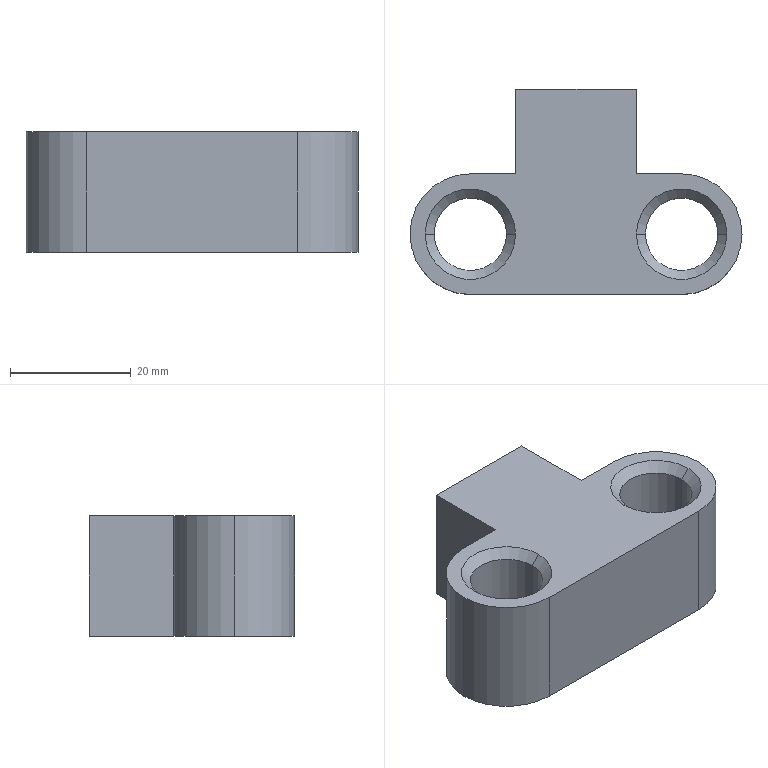Component | SolidWorks | ACQ40x30SB(0)+()-1_ZTDJ-L-400-04-24-MaterialPortBagClamp-T-shapedConnectingRod-2 | 1 solid | 27 faces | box 55 x 34 x 20 mm | volume 17034 mm3 | cone 10 | cylinder 9 | plane 8 | commonest cylinder face diameters 12 x4 20 x3 14 x2 | material 1023 Carbon Steel Sheet (SS)
build123d program:
from build123d import *

# Parameters (mm, degrees)
SKETCH1_R                  = 6
BOSS_EXTRUDE1_DEPTH        = 10
SKETCH4_W                  = 20
SKETCH4_H                  = 20
BOSS_EXTRUDE2_DEPTH        = 14
M14X1_5_TAPPED_HOLE1_D     = 14
M14X1_5_TAPPED_HOLE1_DEPTH = 25.5
M14X1_5_TAPPED_HOLE1_TIP   = 4.206
CHAMFER1_SIZE              = 1.5


with BuildPart() as part:
    # Sketch1 → Boss-Extrude1 (new, symmetric)
    with BuildSketch(Plane.XY):
        with BuildLine():
            Line((-17.5, 10), (17.5, 10))
            ThreePointArc((17.5, 10), (27.5, 0), (17.5, -10))
            Line((17.5, -10), (-17.5, -10))
            ThreePointArc((-17.5, -10), (-27.5, 0), (-17.5, 10))
        make_face()
        with Locations((17.5, 0)):
            Circle(SKETCH1_R, mode=Mode.SUBTRACT)
        with Locations((-17.5, 0)):
            Circle(SKETCH1_R, mode=Mode.SUBTRACT)
    extrude(amount=BOSS_EXTRUDE1_DEPTH, both=True)

    # Sketch4 → Boss-Extrude2 (add)
    with BuildSketch(Plane(origin=(0, 10, 0), x_dir=(1, 0, 0), z_dir=(0, 1, 0))):
        Rectangle(SKETCH4_W, SKETCH4_H)
    extrude(amount=BOSS_EXTRUDE2_DEPTH)

    # M14x1.5 Tapped Hole1
    with Locations(Plane(origin=(0, 24, 0), x_dir=(1, 0, 0), z_dir=(0, 1, 0))):
        with Locations((0, 0)):
            Hole(M14X1_5_TAPPED_HOLE1_D / 2, depth=M14X1_5_TAPPED_HOLE1_DEPTH)
            with Locations((0, 0, -(M14X1_5_TAPPED_HOLE1_DEPTH + M14X1_5_TAPPED_HOLE1_TIP / 2))):  # 118° drill point
                Cone(0, M14X1_5_TAPPED_HOLE1_D / 2, M14X1_5_TAPPED_HOLE1_TIP, mode=Mode.SUBTRACT)

    # Chamfer1
    chamfer1_edges = [part.edges().sort_by_distance(p)[0] for p in [
        (11.5, 0, -10),
        (11.5, 0, 10),
        (-23.5, 0, -10),
        (-23.5, 0, 10),
    ]]
    chamfer(chamfer1_edges, length=CHAMFER1_SIZE)


solid = part.part

# Placed as in the assembly
solid = solid.moved(Location((-28.439, -84.245, 290), (0, 0, 0)))
STEP:
#1=COLOUR_RGB('',0.7922,0.8196,0.9333);
#2=FILL_AREA_STYLE_COLOUR('',#1);
#3=FILL_AREA_STYLE('',(#2));
#4=SURFACE_STYLE_FILL_AREA(#3);
#5=SURFACE_SIDE_STYLE('',(#4));
#6=SURFACE_STYLE_USAGE(.BOTH.,#5);
#7=PRESENTATION_STYLE_ASSIGNMENT((#6));
#8=CARTESIAN_POINT('',(-0.6669,-3.317,11.752));
#9=VERTEX_POINT('',#8);
#10=CARTESIAN_POINT('',(-0.1944,-3.317,11.752));
#11=VERTEX_POINT('',#10);
#12=CARTESIAN_POINT('',(-0.4307,-3.317,11.752));
#13=DIRECTION('',(0.,0.,1.));
#14=DIRECTION('',(1.,0.,0.));
#15=AXIS2_PLACEMENT_3D('',#12,#13,#14);
#16=CIRCLE('',#15,0.2362);
#17=EDGE_CURVE('',#9,#11,#16,.T.);
#18=ORIENTED_EDGE('',*,*,#17,.F.);
#19=CARTESIAN_POINT('',(-0.7259,-3.317,11.811));
#20=VERTEX_POINT('',#19);
#21=CARTESIAN_POINT('',(-0.6669,-3.317,11.752));
#22=DIRECTION('',(-0.7071,0.,0.7071));
#23=VECTOR('',#22,39.37);
#24=LINE('',#21,#23);
#25=EDGE_CURVE('',#9,#20,#24,.T.);
#26=ORIENTED_EDGE('',*,*,#25,.T.);
#27=CARTESIAN_POINT('',(-0.1354,-3.317,11.811));
#28=VERTEX_POINT('',#27);
#29=CARTESIAN_POINT('',(-0.4307,-3.317,11.811));
#30=DIRECTION('',(0.,0.,-1.));
#31=DIRECTION('',(1.,0.,0.));
#32=AXIS2_PLACEMENT_3D('',#29,#30,#31);
#33=CIRCLE('',#32,0.2953);
#34=EDGE_CURVE('',#28,#20,#33,.T.);
#35=ORIENTED_EDGE('',*,*,#34,.F.);
#36=CARTESIAN_POINT('',(-0.1944,-3.317,11.752));
#37=DIRECTION('',(0.7071,0.,0.7071));
#38=VECTOR('',#37,39.37);
#39=LINE('',#36,#38);
#40=EDGE_CURVE('',#11,#28,#39,.T.);
#41=ORIENTED_EDGE('',*,*,#40,.F.);
#42=EDGE_LOOP('',(#18,#26,#35,#41));
#43=FACE_OUTER_BOUND('',#42,.T.);
#44=CARTESIAN_POINT('',(-0.4307,-3.317,11.752));
#45=DIRECTION('',(0.,0.,1.));
#46=DIRECTION('',(1.,0.,0.));
#47=AXIS2_PLACEMENT_3D('',#44,#45,#46);
#48=CONICAL_SURFACE('',#47,0.2362,0.7854);
#49=ADVANCED_FACE('',(#43),#48,.F.);
#50=CARTESIAN_POINT('',(-2.045,-3.317,11.752));
#51=VERTEX_POINT('',#50);
#52=CARTESIAN_POINT('',(-1.572,-3.317,11.752));
#53=VERTEX_POINT('',#52);
#54=CARTESIAN_POINT('',(-1.809,-3.317,11.752));
#55=DIRECTION('',(0.,0.,1.));
#56=DIRECTION('',(1.,0.,0.));
#57=AXIS2_PLACEMENT_3D('',#54,#55,#56);
#58=CIRCLE('',#57,0.2362);
#59=EDGE_CURVE('',#51,#53,#58,.T.);
#60=ORIENTED_EDGE('',*,*,#59,.F.);
#61=CARTESIAN_POINT('',(-2.104,-3.317,11.811));
#62=VERTEX_POINT('',#61);
#63=CARTESIAN_POINT('',(-2.045,-3.317,11.752));
#64=DIRECTION('',(-0.7071,0.,0.7071));
#65=VECTOR('',#64,39.37);
#66=LINE('',#63,#65);
#67=EDGE_CURVE('',#51,#62,#66,.T.);
#68=ORIENTED_EDGE('',*,*,#67,.T.);
#69=CARTESIAN_POINT('',(-1.513,-3.317,11.811));
#70=VERTEX_POINT('',#69);
#71=CARTESIAN_POINT('',(-1.809,-3.317,11.811));
#72=DIRECTION('',(0.,0.,-1.));
#73=DIRECTION('',(1.,0.,0.));
#74=AXIS2_PLACEMENT_3D('',#71,#72,#73);
#75=CIRCLE('',#74,0.2953);
#76=EDGE_CURVE('',#70,#62,#75,.T.);
#77=ORIENTED_EDGE('',*,*,#76,.F.);
#78=CARTESIAN_POINT('',(-1.572,-3.317,11.752));
#79=DIRECTION('',(0.7071,0.,0.7071));
#80=VECTOR('',#79,39.37);
#81=LINE('',#78,#80);
#82=EDGE_CURVE('',#53,#70,#81,.T.);
#83=ORIENTED_EDGE('',*,*,#82,.F.);
#84=EDGE_LOOP('',(#60,#68,#77,#83));
#85=FACE_OUTER_BOUND('',#84,.T.);
#86=CARTESIAN_POINT('',(-1.809,-3.317,11.752));
#87=DIRECTION('',(0.,0.,1.));
#88=DIRECTION('',(1.,0.,0.));
#89=AXIS2_PLACEMENT_3D('',#86,#87,#88);
#90=CONICAL_SURFACE('',#89,0.2362,0.7854);
#91=ADVANCED_FACE('',(#85),#90,.F.);
#92=CARTESIAN_POINT('',(-0.1944,-3.317,11.083));
#93=VERTEX_POINT('',#92);
#94=CARTESIAN_POINT('',(-0.6669,-3.317,11.083));
#95=VERTEX_POINT('',#94);
#96=CARTESIAN_POINT('',(-0.4307,-3.317,11.083));
#97=DIRECTION('',(0.,0.,-1.));
#98=DIRECTION('',(1.,0.,0.));
#99=AXIS2_PLACEMENT_3D('',#96,#97,#98);
#100=CIRCLE('',#99,0.2362);
#101=EDGE_CURVE('',#93,#95,#100,.T.);
#102=ORIENTED_EDGE('',*,*,#101,.F.);
#103=CARTESIAN_POINT('',(-0.1354,-3.317,11.024));
#104=VERTEX_POINT('',#103);
#105=CARTESIAN_POINT('',(-0.1354,-3.317,11.024));
#106=DIRECTION('',(0.7071,0.,-0.7071));
#107=VECTOR('',#106,39.37);
#108=LINE('',#105,#107);
#109=EDGE_CURVE('',#93,#104,#108,.T.);
#110=ORIENTED_EDGE('',*,*,#109,.T.);
#111=CARTESIAN_POINT('',(-0.7259,-3.317,11.024));
#112=VERTEX_POINT('',#111);
#113=CARTESIAN_POINT('',(-0.4307,-3.317,11.024));
#114=DIRECTION('',(0.,0.,1.));
#115=DIRECTION('',(1.,0.,0.));
#116=AXIS2_PLACEMENT_3D('',#113,#114,#115);
#117=CIRCLE('',#116,0.2953);
#118=EDGE_CURVE('',#112,#104,#117,.T.);
#119=ORIENTED_EDGE('',*,*,#118,.F.);
#120=CARTESIAN_POINT('',(-0.7259,-3.317,11.024));
#121=DIRECTION('',(-0.7071,0.,-0.7071));
#122=VECTOR('',#121,39.37);
#123=LINE('',#120,#122);
#124=EDGE_CURVE('',#95,#112,#123,.T.);
#125=ORIENTED_EDGE('',*,*,#124,.F.);
#126=EDGE_LOOP('',(#102,#110,#119,#125));
#127=FACE_OUTER_BOUND('',#126,.T.);
#128=CARTESIAN_POINT('',(-0.4307,-3.317,11.024));
#129=DIRECTION('',(0.,0.,-1.));
#130=DIRECTION('',(-1.,0.,0.));
#131=AXIS2_PLACEMENT_3D('',#128,#129,#130);
#132=CONICAL_SURFACE('',#131,0.2953,0.7854);
#133=ADVANCED_FACE('',(#127),#132,.F.);
#134=CARTESIAN_POINT('',(-1.572,-3.317,11.083));
#135=VERTEX_POINT('',#134);
#136=CARTESIAN_POINT('',(-2.045,-3.317,11.083));
#137=VERTEX_POINT('',#136);
#138=CARTESIAN_POINT('',(-1.809,-3.317,11.083));
#139=DIRECTION('',(0.,0.,-1.));
#140=DIRECTION('',(1.,0.,0.));
#141=AXIS2_PLACEMENT_3D('',#138,#139,#140);
#142=CIRCLE('',#141,0.2362);
#143=EDGE_CURVE('',#135,#137,#142,.T.);
#144=ORIENTED_EDGE('',*,*,#143,.F.);
#145=CARTESIAN_POINT('',(-1.513,-3.317,11.024));
#146=VERTEX_POINT('',#145);
#147=CARTESIAN_POINT('',(-1.513,-3.317,11.024));
#148=DIRECTION('',(0.7071,0.,-0.7071));
#149=VECTOR('',#148,39.37);
#150=LINE('',#147,#149);
#151=EDGE_CURVE('',#135,#146,#150,.T.);
#152=ORIENTED_EDGE('',*,*,#151,.T.);
#153=CARTESIAN_POINT('',(-2.104,-3.317,11.024));
#154=VERTEX_POINT('',#153);
#155=CARTESIAN_POINT('',(-1.809,-3.317,11.024));
#156=DIRECTION('',(0.,0.,1.));
#157=DIRECTION('',(1.,0.,0.));
#158=AXIS2_PLACEMENT_3D('',#155,#156,#157);
#159=CIRCLE('',#158,0.2953);
#160=EDGE_CURVE('',#154,#146,#159,.T.);
#161=ORIENTED_EDGE('',*,*,#160,.F.);
#162=CARTESIAN_POINT('',(-2.104,-3.317,11.024));
#163=DIRECTION('',(-0.7071,0.,-0.7071));
#164=VECTOR('',#163,39.37);
#165=LINE('',#162,#164);
#166=EDGE_CURVE('',#137,#154,#165,.T.);
#167=ORIENTED_EDGE('',*,*,#166,.F.);
#168=EDGE_LOOP('',(#144,#152,#161,#167));
#169=FACE_OUTER_BOUND('',#168,.T.);
#170=CARTESIAN_POINT('',(-1.809,-3.317,11.024));
#171=DIRECTION('',(0.,0.,-1.));
#172=DIRECTION('',(-1.,0.,0.));
#173=AXIS2_PLACEMENT_3D('',#170,#171,#172);
#174=CONICAL_SURFACE('',#173,0.2953,0.7854);
#175=ADVANCED_FACE('',(#169),#174,.F.);
#176=CARTESIAN_POINT('',(-1.12,-3.376,11.142));
#177=VERTEX_POINT('',#176);
#178=CARTESIAN_POINT('',(-1.12,-3.376,11.693));
#179=VERTEX_POINT('',#178);
#180=CARTESIAN_POINT('',(-1.12,-3.376,11.417));
#181=DIRECTION('',(0.,1.,0.));
#182=DIRECTION('',(0.,0.,1.));
#183=AXIS2_PLACEMENT_3D('',#180,#181,#182);
#184=CIRCLE('',#183,0.2756);
#185=EDGE_CURVE('',#177,#179,#184,.T.);
#186=ORIENTED_EDGE('',*,*,#185,.F.);
#187=CARTESIAN_POINT('',(-1.12,-2.372,11.142));
#188=VERTEX_POINT('',#187);
#189=CARTESIAN_POINT('',(-1.12,-2.372,11.142));
#190=DIRECTION('',(0.,1.,0.));
#191=VECTOR('',#190,39.37);
#192=LINE('',#189,#191);
#193=EDGE_CURVE('',#177,#188,#192,.T.);
#194=ORIENTED_EDGE('',*,*,#193,.T.);
#195=CARTESIAN_POINT('',(-1.12,-2.372,11.693));
#196=VERTEX_POINT('',#195);
#197=CARTESIAN_POINT('',(-1.12,-2.372,11.417));
#198=DIRECTION('',(0.,1.,0.));
#199=DIRECTION('',(0.,0.,1.));
#200=AXIS2_PLACEMENT_3D('',#197,#198,#199);
#201=CIRCLE('',#200,0.2756);
#202=EDGE_CURVE('',#188,#196,#201,.T.);
#203=ORIENTED_EDGE('',*,*,#202,.T.);
#204=CARTESIAN_POINT('',(-1.12,-2.372,11.693));
#205=DIRECTION('',(0.,1.,0.));
#206=VECTOR('',#205,39.37);
#207=LINE('',#204,#206);
#208=EDGE_CURVE('',#179,#196,#207,.T.);
#209=ORIENTED_EDGE('',*,*,#208,.F.);
#210=EDGE_LOOP('',(#186,#194,#203,#209));
#211=FACE_OUTER_BOUND('',#210,.T.);
#212=CARTESIAN_POINT('',(-1.12,-2.372,11.417));
#213=DIRECTION('',(0.,1.,0.));
#214=DIRECTION('',(0.,0.,1.));
#215=AXIS2_PLACEMENT_3D('',#212,#213,#214);
#216=CYLINDRICAL_SURFACE('',#215,0.2756);
#217=ADVANCED_FACE('',(#211),#216,.F.);
#218=CARTESIAN_POINT('',(-1.12,-3.541,11.417));
#219=VERTEX_POINT('',#218);
#220=CARTESIAN_POINT('',(-1.12,-3.376,11.693));
#221=DIRECTION('',(0.,0.515,0.8572));
#222=VECTOR('',#221,39.37);
#223=LINE('',#220,#222);
#224=EDGE_CURVE('',#219,#179,#223,.T.);
#225=ORIENTED_EDGE('',*,*,#224,.F.);
#226=CARTESIAN_POINT('',(-1.12,-3.376,11.142));
#227=DIRECTION('',(0.,0.515,-0.8572));
#228=VECTOR('',#227,39.37);
#229=LINE('',#226,#228);
#230=EDGE_CURVE('',#219,#177,#229,.T.);
#231=ORIENTED_EDGE('',*,*,#230,.T.);
#232=ORIENTED_EDGE('',*,*,#185,.T.);
#233=EDGE_LOOP('',(#225,#231,#232));
#234=FACE_OUTER_BOUND('',#233,.T.);
#235=CARTESIAN_POINT('',(-1.12,-3.376,11.417));
#236=DIRECTION('',(0.,1.,0.));
#237=DIRECTION('',(0.,0.,1.));
#238=AXIS2_PLACEMENT_3D('',#235,#236,#237);
#239=CONICAL_SURFACE('',#238,0.2756,1.03);
#240=ADVANCED_FACE('',(#234),#239,.F.);
#241=ORIENTED_EDGE('',*,*,#59,.T.);
#242=CARTESIAN_POINT('',(-1.572,-3.317,11.811));
#243=DIRECTION('',(0.,0.,-1.));
#244=VECTOR('',#243,39.37);
#245=LINE('',#242,#244);
#246=EDGE_CURVE('',#53,#135,#245,.T.);
#247=ORIENTED_EDGE('',*,*,#246,.T.);
#248=ORIENTED_EDGE('',*,*,#143,.T.);
#249=CARTESIAN_POINT('',(-2.045,-3.317,11.811));
#250=DIRECTION('',(0.,0.,-1.));
#251=VECTOR('',#250,39.37);
#252=LINE('',#249,#251);
#253=EDGE_CURVE('',#51,#137,#252,.T.);
#254=ORIENTED_EDGE('',*,*,#253,.F.);
#255=EDGE_LOOP('',(#241,#247,#248,#254));
#256=FACE_OUTER_BOUND('',#255,.T.);
#257=CARTESIAN_POINT('',(-1.809,-3.317,11.811));
#258=DIRECTION('',(0.,0.,-1.));
#259=DIRECTION('',(-1.,0.,0.));
#260=AXIS2_PLACEMENT_3D('',#257,#258,#259);
#261=CYLINDRICAL_SURFACE('',#260,0.2362);
#262=ADVANCED_FACE('',(#256),#261,.F.);
#263=ORIENTED_EDGE('',*,*,#17,.T.);
#264=CARTESIAN_POINT('',(-0.1944,-3.317,11.811));
#265=DIRECTION('',(0.,0.,-1.));
#266=VECTOR('',#265,39.37);
#267=LINE('',#264,#266);
#268=EDGE_CURVE('',#11,#93,#267,.T.);
#269=ORIENTED_EDGE('',*,*,#268,.T.);
#270=ORIENTED_EDGE('',*,*,#101,.T.);
#271=CARTESIAN_POINT('',(-0.6669,-3.317,11.811));
#272=DIRECTION('',(0.,0.,-1.));
#273=VECTOR('',#272,39.37);
#274=LINE('',#271,#273);
#275=EDGE_CURVE('',#9,#95,#274,.T.);
#276=ORIENTED_EDGE('',*,*,#275,.F.);
#277=EDGE_LOOP('',(#263,#269,#270,#276));
#278=FACE_OUTER_BOUND('',#277,.T.);
#279=CARTESIAN_POINT('',(-0.4307,-3.317,11.811));
#280=DIRECTION('',(0.,0.,-1.));
#281=DIRECTION('',(-1.,0.,0.));
#282=AXIS2_PLACEMENT_3D('',#279,#280,#281);
#283=CYLINDRICAL_SURFACE('',#282,0.2362);
#284=ADVANCED_FACE('',(#278),#283,.F.);
#285=CARTESIAN_POINT('',(-2.202,-3.317,11.811));
#286=VERTEX_POINT('',#285);
#287=CARTESIAN_POINT('',(-1.809,-3.71,11.811));
#288=VERTEX_POINT('',#287);
#289=CARTESIAN_POINT('',(-1.809,-3.317,11.811));
#290=DIRECTION('',(0.,0.,1.));
#291=DIRECTION('',(1.,0.,0.));
#292=AXIS2_PLACEMENT_3D('',#289,#290,#291);
#293=CIRCLE('',#292,0.3937);
#294=EDGE_CURVE('',#286,#288,#293,.T.);
#295=ORIENTED_EDGE('',*,*,#294,.F.);
#296=CARTESIAN_POINT('',(-2.202,-3.317,11.024));
#297=VERTEX_POINT('',#296);
#298=CARTESIAN_POINT('',(-2.202,-3.317,11.811));
#299=DIRECTION('',(0.,0.,-1.));
#300=VECTOR('',#299,39.37);
#301=LINE('',#298,#300);
#302=EDGE_CURVE('',#286,#297,#301,.T.);
#303=ORIENTED_EDGE('',*,*,#302,.T.);
#304=CARTESIAN_POINT('',(-1.809,-3.71,11.024));
#305=VERTEX_POINT('',#304);
#306=CARTESIAN_POINT('',(-1.809,-3.317,11.024));
#307=DIRECTION('',(0.,0.,1.));
#308=DIRECTION('',(1.,0.,0.));
#309=AXIS2_PLACEMENT_3D('',#306,#307,#308);
#310=CIRCLE('',#309,0.3937);
#311=EDGE_CURVE('',#297,#305,#310,.T.);
#312=ORIENTED_EDGE('',*,*,#311,.T.);
#313=CARTESIAN_POINT('',(-1.809,-3.71,11.811));
#314=DIRECTION('',(0.,0.,-1.));
#315=VECTOR('',#314,39.37);
#316=LINE('',#313,#315);
#317=EDGE_CURVE('',#288,#305,#316,.T.);
#318=ORIENTED_EDGE('',*,*,#317,.F.);
#319=EDGE_LOOP('',(#295,#303,#312,#318));
#320=FACE_OUTER_BOUND('',#319,.T.);
#321=CARTESIAN_POINT('',(-1.809,-3.317,11.811));
#322=DIRECTION('',(0.,0.,-1.));
#323=DIRECTION('',(-1.,0.,0.));
#324=AXIS2_PLACEMENT_3D('',#321,#322,#323);
#325=CYLINDRICAL_SURFACE('',#324,0.3937);
#326=ADVANCED_FACE('',(#320),#325,.T.);
#327=CARTESIAN_POINT('',(-0.7259,-2.923,11.811));
#328=VERTEX_POINT('',#327);
#329=CARTESIAN_POINT('',(-0.7259,-2.923,11.024));
#330=VERTEX_POINT('',#329);
#331=CARTESIAN_POINT('',(-0.7259,-2.923,11.811));
#332=DIRECTION('',(0.,0.,-1.));
#333=VECTOR('',#332,39.37);
#334=LINE('',#331,#333);
#335=EDGE_CURVE('',#328,#330,#334,.T.);
#336=ORIENTED_EDGE('',*,*,#335,.F.);
#337=CARTESIAN_POINT('',(-0.4307,-2.923,11.811));
#338=VERTEX_POINT('',#337);
#339=CARTESIAN_POINT('',(-1.809,-2.923,11.811));
#340=DIRECTION('',(-1.,-0.,0.));
#341=VECTOR('',#340,39.37);
#342=LINE('',#339,#341);
#343=EDGE_CURVE('',#338,#328,#342,.T.);
#344=ORIENTED_EDGE('',*,*,#343,.F.);
#345=CARTESIAN_POINT('',(-0.4307,-2.923,11.024));
#346=VERTEX_POINT('',#345);
#347=CARTESIAN_POINT('',(-0.4307,-2.923,11.811));
#348=DIRECTION('',(0.,0.,-1.));
#349=VECTOR('',#348,39.37);
#350=LINE('',#347,#349);
#351=EDGE_CURVE('',#338,#346,#350,.T.);
#352=ORIENTED_EDGE('',*,*,#351,.T.);
#353=CARTESIAN_POINT('',(-1.809,-2.923,11.024));
#354=DIRECTION('',(-1.,-0.,0.));
#355=VECTOR('',#354,39.37);
#356=LINE('',#353,#355);
#357=EDGE_CURVE('',#346,#330,#356,.T.);
#358=ORIENTED_EDGE('',*,*,#357,.T.);
#359=EDGE_LOOP('',(#336,#344,#352,#358));
#360=FACE_OUTER_BOUND('',#359,.T.);
#361=CARTESIAN_POINT('',(-1.809,-2.923,11.811));
#362=DIRECTION('',(0.,-1.,0.));
#363=DIRECTION('',(1.,0.,0.));
#364=AXIS2_PLACEMENT_3D('',#361,#362,#363);
#365=PLANE('',#364);
#366=ADVANCED_FACE('',(#360),#365,.F.);
#367=CARTESIAN_POINT('',(-1.513,-2.923,11.024));
#368=VERTEX_POINT('',#367);
#369=CARTESIAN_POINT('',(-1.513,-2.923,11.811));
#370=VERTEX_POINT('',#369);
#371=CARTESIAN_POINT('',(-1.513,-2.923,11.811));
#372=DIRECTION('',(0.,0.,1.));
#373=VECTOR('',#372,39.37);
#374=LINE('',#371,#373);
#375=EDGE_CURVE('',#368,#370,#374,.T.);
#376=ORIENTED_EDGE('',*,*,#375,.F.);
#377=CARTESIAN_POINT('',(-1.809,-2.923,11.024));
#378=VERTEX_POINT('',#377);
#379=CARTESIAN_POINT('',(-1.809,-2.923,11.024));
#380=DIRECTION('',(-1.,-0.,0.));
#381=VECTOR('',#380,39.37);
#382=LINE('',#379,#381);
#383=EDGE_CURVE('',#368,#378,#382,.T.);
#384=ORIENTED_EDGE('',*,*,#383,.T.);
#385=CARTESIAN_POINT('',(-1.809,-2.923,11.811));
#386=VERTEX_POINT('',#385);
#387=CARTESIAN_POINT('',(-1.809,-2.923,11.811));
#388=DIRECTION('',(0.,0.,-1.));
#389=VECTOR('',#388,39.37);
#390=LINE('',#387,#389);
#391=EDGE_CURVE('',#386,#378,#390,.T.);
#392=ORIENTED_EDGE('',*,*,#391,.F.);
#393=CARTESIAN_POINT('',(-1.809,-2.923,11.811));
#394=DIRECTION('',(-1.,-0.,0.));
#395=VECTOR('',#394,39.37);
#396=LINE('',#393,#395);
#397=EDGE_CURVE('',#370,#386,#396,.T.);
#398=ORIENTED_EDGE('',*,*,#397,.F.);
#399=EDGE_LOOP('',(#376,#384,#392,#398));
#400=FACE_OUTER_BOUND('',#399,.T.);
#401=CARTESIAN_POINT('',(-1.809,-2.923,11.811));
#402=DIRECTION('',(0.,-1.,0.));
#403=DIRECTION('',(1.,0.,0.));
#404=AXIS2_PLACEMENT_3D('',#401,#402,#403);
#405=PLANE('',#404);
#406=ADVANCED_FACE('',(#400),#405,.F.);
#407=ORIENTED_EDGE('',*,*,#76,.T.);
#408=CARTESIAN_POINT('',(-1.809,-3.317,11.811));
#409=DIRECTION('',(0.,0.,-1.));
#410=DIRECTION('',(1.,0.,0.));
#411=AXIS2_PLACEMENT_3D('',#408,#409,#410);
#412=CIRCLE('',#411,0.2953);
#413=EDGE_CURVE('',#62,#70,#412,.T.);
#414=ORIENTED_EDGE('',*,*,#413,.T.);
#415=EDGE_LOOP('',(#407,#414));
#416=FACE_BOUND('',#415,.T.);
#417=ORIENTED_EDGE('',*,*,#34,.T.);
#418=CARTESIAN_POINT('',(-0.4307,-3.317,11.811));
#419=DIRECTION('',(0.,0.,-1.));
#420=DIRECTION('',(1.,0.,0.));
#421=AXIS2_PLACEMENT_3D('',#418,#419,#420);
#422=CIRCLE('',#421,0.2953);
#423=EDGE_CURVE('',#20,#28,#422,.T.);
#424=ORIENTED_EDGE('',*,*,#423,.T.);
#425=EDGE_LOOP('',(#417,#424));
#426=FACE_BOUND('',#425,.T.);
#427=CARTESIAN_POINT('',(-1.809,-3.317,11.811));
#428=DIRECTION('',(0.,0.,1.));
#429=DIRECTION('',(1.,0.,0.));
#430=AXIS2_PLACEMENT_3D('',#427,#428,#429);
#431=CIRCLE('',#430,0.3937);
#432=EDGE_CURVE('',#386,#286,#431,.T.);
#433=ORIENTED_EDGE('',*,*,#432,.T.);
#434=ORIENTED_EDGE('',*,*,#294,.T.);
#435=CARTESIAN_POINT('',(-0.4307,-3.71,11.811));
#436=VERTEX_POINT('',#435);
#437=CARTESIAN_POINT('',(-1.809,-3.71,11.811));
#438=DIRECTION('',(1.,0.,0.));
#439=VECTOR('',#438,39.37);
#440=LINE('',#437,#439);
#441=EDGE_CURVE('',#288,#436,#440,.T.);
#442=ORIENTED_EDGE('',*,*,#441,.T.);
#443=CARTESIAN_POINT('',(-0.4307,-3.317,11.811));
#444=DIRECTION('',(0.,0.,1.));
#445=DIRECTION('',(1.,0.,0.));
#446=AXIS2_PLACEMENT_3D('',#443,#444,#445);
#447=CIRCLE('',#446,0.3937);
#448=EDGE_CURVE('',#436,#338,#447,.T.);
#449=ORIENTED_EDGE('',*,*,#448,.T.);
#450=ORIENTED_EDGE('',*,*,#343,.T.);
#451=CARTESIAN_POINT('',(-0.7259,-2.372,11.811));
#452=VERTEX_POINT('',#451);
#453=CARTESIAN_POINT('',(-0.7259,-2.372,11.811));
#454=DIRECTION('',(0.,-1.,0.));
#455=VECTOR('',#454,39.37);
#456=LINE('',#453,#455);
#457=EDGE_CURVE('',#452,#328,#456,.T.);
#458=ORIENTED_EDGE('',*,*,#457,.F.);
#459=CARTESIAN_POINT('',(-1.513,-2.372,11.811));
#460=VERTEX_POINT('',#459);
#461=CARTESIAN_POINT('',(-1.513,-2.372,11.811));
#462=DIRECTION('',(1.,0.,0.));
#463=VECTOR('',#462,39.37);
#464=LINE('',#461,#463);
#465=EDGE_CURVE('',#460,#452,#464,.T.);
#466=ORIENTED_EDGE('',*,*,#465,.F.);
#467=CARTESIAN_POINT('',(-1.513,-2.372,11.811));
#468=DIRECTION('',(0.,-1.,0.));
#469=VECTOR('',#468,39.37);
#470=LINE('',#467,#469);
#471=EDGE_CURVE('',#460,#370,#470,.T.);
#472=ORIENTED_EDGE('',*,*,#471,.T.);
#473=ORIENTED_EDGE('',*,*,#397,.T.);
#474=EDGE_LOOP('',(#433,#434,#442,#449,#450,#458,#466,#472,#473));
#475=FACE_OUTER_BOUND('',#474,.T.);
#476=CARTESIAN_POINT('',(-1.809,-3.317,11.811));
#477=DIRECTION('',(0.,0.,1.));
#478=DIRECTION('',(1.,0.,0.));
#479=AXIS2_PLACEMENT_3D('',#476,#477,#478);
#480=PLANE('',#479);
#481=ADVANCED_FACE('',(#416,#426,#475),#480,.T.);
#482=ORIENTED_EDGE('',*,*,#160,.T.);
#483=CARTESIAN_POINT('',(-1.809,-3.317,11.024));
#484=DIRECTION('',(0.,0.,1.));
#485=DIRECTION('',(1.,0.,0.));
#486=AXIS2_PLACEMENT_3D('',#483,#484,#485);
#487=CIRCLE('',#486,0.2953);
#488=EDGE_CURVE('',#146,#154,#487,.T.);
#489=ORIENTED_EDGE('',*,*,#488,.T.);
#490=EDGE_LOOP('',(#482,#489));
#491=FACE_BOUND('',#490,.T.);
#492=ORIENTED_EDGE('',*,*,#118,.T.);
#493=CARTESIAN_POINT('',(-0.4307,-3.317,11.024));
#494=DIRECTION('',(0.,0.,1.));
#495=DIRECTION('',(1.,0.,0.));
#496=AXIS2_PLACEMENT_3D('',#493,#494,#495);
#497=CIRCLE('',#496,0.2953);
#498=EDGE_CURVE('',#104,#112,#497,.T.);
#499=ORIENTED_EDGE('',*,*,#498,.T.);
#500=EDGE_LOOP('',(#492,#499));
#501=FACE_BOUND('',#500,.T.);
#502=CARTESIAN_POINT('',(-1.809,-3.317,11.024));
#503=DIRECTION('',(0.,0.,1.));
#504=DIRECTION('',(1.,0.,0.));
#505=AXIS2_PLACEMENT_3D('',#502,#503,#504);
#506=CIRCLE('',#505,0.3937);
#507=EDGE_CURVE('',#378,#297,#506,.T.);
#508=ORIENTED_EDGE('',*,*,#507,.F.);
#509=ORIENTED_EDGE('',*,*,#383,.F.);
#510=CARTESIAN_POINT('',(-1.513,-2.372,11.024));
#511=VERTEX_POINT('',#510);
#512=CARTESIAN_POINT('',(-1.513,-2.372,11.024));
#513=DIRECTION('',(0.,-1.,0.));
#514=VECTOR('',#513,39.37);
#515=LINE('',#512,#514);
#516=EDGE_CURVE('',#511,#368,#515,.T.);
#517=ORIENTED_EDGE('',*,*,#516,.F.);
#518=CARTESIAN_POINT('',(-0.7259,-2.372,11.024));
#519=VERTEX_POINT('',#518);
#520=CARTESIAN_POINT('',(-1.513,-2.372,11.024));
#521=DIRECTION('',(-1.,-0.,0.));
#522=VECTOR('',#521,39.37);
#523=LINE('',#520,#522);
#524=EDGE_CURVE('',#519,#511,#523,.T.);
#525=ORIENTED_EDGE('',*,*,#524,.F.);
#526=CARTESIAN_POINT('',(-0.7259,-2.372,11.024));
#527=DIRECTION('',(0.,-1.,0.));
#528=VECTOR('',#527,39.37);
#529=LINE('',#526,#528);
#530=EDGE_CURVE('',#519,#330,#529,.T.);
#531=ORIENTED_EDGE('',*,*,#530,.T.);
#532=ORIENTED_EDGE('',*,*,#357,.F.);
#533=CARTESIAN_POINT('',(-0.4307,-3.71,11.024));
#534=VERTEX_POINT('',#533);
#535=CARTESIAN_POINT('',(-0.4307,-3.317,11.024));
#536=DIRECTION('',(0.,0.,1.));
#537=DIRECTION('',(1.,0.,0.));
#538=AXIS2_PLACEMENT_3D('',#535,#536,#537);
#539=CIRCLE('',#538,0.3937);
#540=EDGE_CURVE('',#534,#346,#539,.T.);
#541=ORIENTED_EDGE('',*,*,#540,.F.);
#542=CARTESIAN_POINT('',(-1.809,-3.71,11.024));
#543=DIRECTION('',(1.,0.,0.));
#544=VECTOR('',#543,39.37);
#545=LINE('',#542,#544);
#546=EDGE_CURVE('',#305,#534,#545,.T.);
#547=ORIENTED_EDGE('',*,*,#546,.F.);
#548=ORIENTED_EDGE('',*,*,#311,.F.);
#549=EDGE_LOOP('',(#508,#509,#517,#525,#531,#532,#541,#547,#548));
#550=FACE_OUTER_BOUND('',#549,.T.);
#551=CARTESIAN_POINT('',(-1.809,-3.317,11.024));
#552=DIRECTION('',(0.,0.,1.));
#553=DIRECTION('',(1.,0.,0.));
#554=AXIS2_PLACEMENT_3D('',#551,#552,#553);
#555=PLANE('',#554);
#556=ADVANCED_FACE('',(#491,#501,#550),#555,.F.);
#557=ORIENTED_EDGE('',*,*,#302,.F.);
#558=ORIENTED_EDGE('',*,*,#432,.F.);
#559=ORIENTED_EDGE('',*,*,#391,.T.);
#560=ORIENTED_EDGE('',*,*,#507,.T.);
#561=EDGE_LOOP('',(#557,#558,#559,#560));
#562=FACE_OUTER_BOUND('',#561,.T.);
#563=CARTESIAN_POINT('',(-1.809,-3.317,11.811));
#564=DIRECTION('',(0.,0.,-1.));
#565=DIRECTION('',(-1.,0.,0.));
#566=AXIS2_PLACEMENT_3D('',#563,#564,#565);
#567=CYLINDRICAL_SURFACE('',#566,0.3937);
#568=ADVANCED_FACE('',(#562),#567,.T.);
#569=ORIENTED_EDGE('',*,*,#546,.T.);
#570=CARTESIAN_POINT('',(-0.4307,-3.71,11.811));
#571=DIRECTION('',(0.,0.,-1.));
#572=VECTOR('',#571,39.37);
#573=LINE('',#570,#572);
#574=EDGE_CURVE('',#436,#534,#573,.T.);
#575=ORIENTED_EDGE('',*,*,#574,.F.);
#576=ORIENTED_EDGE('',*,*,#441,.F.);
#577=ORIENTED_EDGE('',*,*,#317,.T.);
#578=EDGE_LOOP('',(#569,#575,#576,#577));
#579=FACE_OUTER_BOUND('',#578,.T.);
#580=CARTESIAN_POINT('',(-1.809,-3.71,11.811));
#581=DIRECTION('',(-0.,1.,0.));
#582=DIRECTION('',(-1.,-0.,0.));
#583=AXIS2_PLACEMENT_3D('',#580,#581,#582);
#584=PLANE('',#583);
#585=ADVANCED_FACE('',(#579),#584,.F.);
#586=ORIENTED_EDGE('',*,*,#540,.T.);
#587=ORIENTED_EDGE('',*,*,#351,.F.);
#588=ORIENTED_EDGE('',*,*,#448,.F.);
#589=ORIENTED_EDGE('',*,*,#574,.T.);
#590=EDGE_LOOP('',(#586,#587,#588,#589));
#591=FACE_OUTER_BOUND('',#590,.T.);
#592=CARTESIAN_POINT('',(-0.4307,-3.317,11.811));
#593=DIRECTION('',(0.,0.,-1.));
#594=DIRECTION('',(-1.,0.,0.));
#595=AXIS2_PLACEMENT_3D('',#592,#593,#594);
#596=CYLINDRICAL_SURFACE('',#595,0.3937);
#597=ADVANCED_FACE('',(#591),#596,.T.);
#598=ORIENTED_EDGE('',*,*,#268,.F.);
#599=CARTESIAN_POINT('',(-0.4307,-3.317,11.752));
#600=DIRECTION('',(0.,0.,1.));
#601=DIRECTION('',(1.,0.,0.));
#602=AXIS2_PLACEMENT_3D('',#599,#600,#601);
#603=CIRCLE('',#602,0.2362);
#604=EDGE_CURVE('',#11,#9,#603,.T.);
#605=ORIENTED_EDGE('',*,*,#604,.T.);
#606=ORIENTED_EDGE('',*,*,#275,.T.);
#607=CARTESIAN_POINT('',(-0.4307,-3.317,11.083));
#608=DIRECTION('',(0.,0.,-1.));
#609=DIRECTION('',(1.,0.,0.));
#610=AXIS2_PLACEMENT_3D('',#607,#608,#609);
#611=CIRCLE('',#610,0.2362);
#612=EDGE_CURVE('',#95,#93,#611,.T.);
#613=ORIENTED_EDGE('',*,*,#612,.T.);
#614=EDGE_LOOP('',(#598,#605,#606,#613));
#615=FACE_OUTER_BOUND('',#614,.T.);
#616=CARTESIAN_POINT('',(-0.4307,-3.317,11.811));
#617=DIRECTION('',(0.,0.,-1.));
#618=DIRECTION('',(-1.,0.,0.));
#619=AXIS2_PLACEMENT_3D('',#616,#617,#618);
#620=CYLINDRICAL_SURFACE('',#619,0.2362);
#621=ADVANCED_FACE('',(#615),#620,.F.);
#622=ORIENTED_EDGE('',*,*,#246,.F.);
#623=CARTESIAN_POINT('',(-1.809,-3.317,11.752));
#624=DIRECTION('',(0.,0.,1.));
#625=DIRECTION('',(1.,0.,0.));
#626=AXIS2_PLACEMENT_3D('',#623,#624,#625);
#627=CIRCLE('',#626,0.2362);
#628=EDGE_CURVE('',#53,#51,#627,.T.);
#629=ORIENTED_EDGE('',*,*,#628,.T.);
#630=ORIENTED_EDGE('',*,*,#253,.T.);
#631=CARTESIAN_POINT('',(-1.809,-3.317,11.083));
#632=DIRECTION('',(0.,0.,-1.));
#633=DIRECTION('',(1.,0.,0.));
#634=AXIS2_PLACEMENT_3D('',#631,#632,#633);
#635=CIRCLE('',#634,0.2362);
#636=EDGE_CURVE('',#137,#135,#635,.T.);
#637=ORIENTED_EDGE('',*,*,#636,.T.);
#638=EDGE_LOOP('',(#622,#629,#630,#637));
#639=FACE_OUTER_BOUND('',#638,.T.);
#640=CARTESIAN_POINT('',(-1.809,-3.317,11.811));
#641=DIRECTION('',(0.,0.,-1.));
#642=DIRECTION('',(-1.,0.,0.));
#643=AXIS2_PLACEMENT_3D('',#640,#641,#642);
#644=CYLINDRICAL_SURFACE('',#643,0.2362);
#645=ADVANCED_FACE('',(#639),#644,.F.);
#646=ORIENTED_EDGE('',*,*,#335,.T.);
#647=ORIENTED_EDGE('',*,*,#530,.F.);
#648=CARTESIAN_POINT('',(-0.7259,-2.372,11.811));
#649=DIRECTION('',(0.,0.,-1.));
#650=VECTOR('',#649,39.37);
#651=LINE('',#648,#650);
#652=EDGE_CURVE('',#452,#519,#651,.T.);
#653=ORIENTED_EDGE('',*,*,#652,.F.);
#654=ORIENTED_EDGE('',*,*,#457,.T.);
#655=EDGE_LOOP('',(#646,#647,#653,#654));
#656=FACE_OUTER_BOUND('',#655,.T.);
#657=CARTESIAN_POINT('',(-0.7259,-2.372,11.811));
#658=DIRECTION('',(-1.,-0.,0.));
#659=DIRECTION('',(0.,-1.,0.));
#660=AXIS2_PLACEMENT_3D('',#657,#658,#659);
#661=PLANE('',#660);
#662=ADVANCED_FACE('',(#656),#661,.F.);
#663=ORIENTED_EDGE('',*,*,#375,.T.);
#664=ORIENTED_EDGE('',*,*,#471,.F.);
#665=CARTESIAN_POINT('',(-1.513,-2.372,11.811));
#666=DIRECTION('',(0.,0.,1.));
#667=VECTOR('',#666,39.37);
#668=LINE('',#665,#667);
#669=EDGE_CURVE('',#511,#460,#668,.T.);
#670=ORIENTED_EDGE('',*,*,#669,.F.);
#671=ORIENTED_EDGE('',*,*,#516,.T.);
#672=EDGE_LOOP('',(#663,#664,#670,#671));
#673=FACE_OUTER_BOUND('',#672,.T.);
#674=CARTESIAN_POINT('',(-1.513,-2.372,11.811));
#675=DIRECTION('',(1.,0.,0.));
#676=DIRECTION('',(-0.,1.,0.));
#677=AXIS2_PLACEMENT_3D('',#674,#675,#676);
#678=PLANE('',#677);
#679=ADVANCED_FACE('',(#673),#678,.F.);
#680=CARTESIAN_POINT('',(-1.12,-2.372,11.417));
#681=DIRECTION('',(0.,1.,0.));
#682=DIRECTION('',(0.,0.,1.));
#683=AXIS2_PLACEMENT_3D('',#680,#681,#682);
#684=CIRCLE('',#683,0.2756);
#685=EDGE_CURVE('',#196,#188,#684,.T.);
#686=ORIENTED_EDGE('',*,*,#685,.F.);
#687=ORIENTED_EDGE('',*,*,#202,.F.);
#688=EDGE_LOOP('',(#686,#687));
#689=FACE_BOUND('',#688,.T.);
#690=ORIENTED_EDGE('',*,*,#652,.T.);
#691=ORIENTED_EDGE('',*,*,#524,.T.);
#692=ORIENTED_EDGE('',*,*,#669,.T.);
#693=ORIENTED_EDGE('',*,*,#465,.T.);
#694=EDGE_LOOP('',(#690,#691,#692,#693));
#695=FACE_OUTER_BOUND('',#694,.T.);
#696=CARTESIAN_POINT('',(-1.12,-2.372,11.417));
#697=DIRECTION('',(0.,-1.,0.));
#698=DIRECTION('',(1.,0.,0.));
#699=AXIS2_PLACEMENT_3D('',#696,#697,#698);
#700=PLANE('',#699);
#701=ADVANCED_FACE('',(#689,#695),#700,.F.);
#702=ORIENTED_EDGE('',*,*,#230,.F.);
#703=ORIENTED_EDGE('',*,*,#224,.T.);
#704=CARTESIAN_POINT('',(-1.12,-3.376,11.417));
#705=DIRECTION('',(0.,1.,0.));
#706=DIRECTION('',(0.,0.,1.));
#707=AXIS2_PLACEMENT_3D('',#704,#705,#706);
#708=CIRCLE('',#707,0.2756);
#709=EDGE_CURVE('',#179,#177,#708,.T.);
#710=ORIENTED_EDGE('',*,*,#709,.T.);
#711=EDGE_LOOP('',(#702,#703,#710));
#712=FACE_OUTER_BOUND('',#711,.T.);
#713=CARTESIAN_POINT('',(-1.12,-3.376,11.417));
#714=DIRECTION('',(0.,1.,0.));
#715=DIRECTION('',(0.,0.,1.));
#716=AXIS2_PLACEMENT_3D('',#713,#714,#715);
#717=CONICAL_SURFACE('',#716,0.2756,1.03);
#718=ADVANCED_FACE('',(#712),#717,.F.);
#719=ORIENTED_EDGE('',*,*,#193,.F.);
#720=ORIENTED_EDGE('',*,*,#709,.F.);
#721=ORIENTED_EDGE('',*,*,#208,.T.);
#722=ORIENTED_EDGE('',*,*,#685,.T.);
#723=EDGE_LOOP('',(#719,#720,#721,#722));
#724=FACE_OUTER_BOUND('',#723,.T.);
#725=CARTESIAN_POINT('',(-1.12,-2.372,11.417));
#726=DIRECTION('',(0.,1.,0.));
#727=DIRECTION('',(0.,0.,1.));
#728=AXIS2_PLACEMENT_3D('',#725,#726,#727);
#729=CYLINDRICAL_SURFACE('',#728,0.2756);
#730=ADVANCED_FACE('',(#724),#729,.F.);
#731=ORIENTED_EDGE('',*,*,#151,.F.);
#732=ORIENTED_EDGE('',*,*,#636,.F.);
#733=ORIENTED_EDGE('',*,*,#166,.T.);
#734=ORIENTED_EDGE('',*,*,#488,.F.);
#735=EDGE_LOOP('',(#731,#732,#733,#734));
#736=FACE_OUTER_BOUND('',#735,.T.);
#737=CARTESIAN_POINT('',(-1.809,-3.317,11.024));
#738=DIRECTION('',(0.,0.,-1.));
#739=DIRECTION('',(-1.,0.,0.));
#740=AXIS2_PLACEMENT_3D('',#737,#738,#739);
#741=CONICAL_SURFACE('',#740,0.2953,0.7854);
#742=ADVANCED_FACE('',(#736),#741,.F.);
#743=ORIENTED_EDGE('',*,*,#109,.F.);
#744=ORIENTED_EDGE('',*,*,#612,.F.);
#745=ORIENTED_EDGE('',*,*,#124,.T.);
#746=ORIENTED_EDGE('',*,*,#498,.F.);
#747=EDGE_LOOP('',(#743,#744,#745,#746));
#748=FACE_OUTER_BOUND('',#747,.T.);
#749=CARTESIAN_POINT('',(-0.4307,-3.317,11.024));
#750=DIRECTION('',(0.,0.,-1.));
#751=DIRECTION('',(-1.,0.,0.));
#752=AXIS2_PLACEMENT_3D('',#749,#750,#751);
#753=CONICAL_SURFACE('',#752,0.2953,0.7854);
#754=ADVANCED_FACE('',(#748),#753,.F.);
#755=ORIENTED_EDGE('',*,*,#67,.F.);
#756=ORIENTED_EDGE('',*,*,#628,.F.);
#757=ORIENTED_EDGE('',*,*,#82,.T.);
#758=ORIENTED_EDGE('',*,*,#413,.F.);
#759=EDGE_LOOP('',(#755,#756,#757,#758));
#760=FACE_OUTER_BOUND('',#759,.T.);
#761=CARTESIAN_POINT('',(-1.809,-3.317,11.752));
#762=DIRECTION('',(0.,0.,1.));
#763=DIRECTION('',(1.,0.,0.));
#764=AXIS2_PLACEMENT_3D('',#761,#762,#763);
#765=CONICAL_SURFACE('',#764,0.2362,0.7854);
#766=ADVANCED_FACE('',(#760),#765,.F.);
#767=ORIENTED_EDGE('',*,*,#25,.F.);
#768=ORIENTED_EDGE('',*,*,#604,.F.);
#769=ORIENTED_EDGE('',*,*,#40,.T.);
#770=ORIENTED_EDGE('',*,*,#423,.F.);
#771=EDGE_LOOP('',(#767,#768,#769,#770));
#772=FACE_OUTER_BOUND('',#771,.T.);
#773=CARTESIAN_POINT('',(-0.4307,-3.317,11.752));
#774=DIRECTION('',(0.,0.,1.));
#775=DIRECTION('',(1.,0.,0.));
#776=AXIS2_PLACEMENT_3D('',#773,#774,#775);
#777=CONICAL_SURFACE('',#776,0.2362,0.7854);
#778=ADVANCED_FACE('',(#772),#777,.F.);
#779=CLOSED_SHELL('',(#49,#91,#133,#175,#217,#240,#262,#284,#326,#366,#406,#481,#556,#568,#585,#597,#621,#645,#662,#679,#701,#718,#730,#742,#754,#766,#778));
#780=MANIFOLD_SOLID_BREP('',#779);
#781=STYLED_ITEM('',(#7),#780);
#782=(LENGTH_UNIT()NAMED_UNIT(*)SI_UNIT($,.METRE.));
#783=LENGTH_MEASURE_WITH_UNIT(LENGTH_MEASURE(0.0254),#782);
#784=DIMENSIONAL_EXPONENTS(1.,0.,0.,0.,0.,0.,0.);
#785=(CONVERSION_BASED_UNIT('',#783)LENGTH_UNIT()NAMED_UNIT(#784));
#786=UNCERTAINTY_MEASURE_WITH_UNIT(LENGTH_MEASURE(0.00001),#785,'','');
#787=(NAMED_UNIT(*)PLANE_ANGLE_UNIT()SI_UNIT($,.RADIAN.));
#788=(NAMED_UNIT(*)SI_UNIT($,.STERADIAN.)SOLID_ANGLE_UNIT());
#789=(GEOMETRIC_REPRESENTATION_CONTEXT(3)GLOBAL_UNCERTAINTY_ASSIGNED_CONTEXT((#786))GLOBAL_UNIT_ASSIGNED_CONTEXT((#785,#787,#788))REPRESENTATION_CONTEXT('',''));
#790=MECHANICAL_DESIGN_GEOMETRIC_PRESENTATION_REPRESENTATION('',(#781),#789);
#791=PRESENTATION_LAYER_ASSIGNMENT('','',(#781));
#792=CARTESIAN_POINT('',(0.,0.,0.));
#793=DIRECTION('',(0.,0.,1.));
#794=DIRECTION('',(1.,0.,0.));
#795=AXIS2_PLACEMENT_3D('',#792,#793,#794);
#796=(LENGTH_UNIT()NAMED_UNIT(*)SI_UNIT($,.METRE.));
#797=LENGTH_MEASURE_WITH_UNIT(LENGTH_MEASURE(0.0254),#796);
#798=DIMENSIONAL_EXPONENTS(1.,0.,0.,0.,0.,0.,0.);
#799=(CONVERSION_BASED_UNIT('',#797)LENGTH_UNIT()NAMED_UNIT(#798));
#800=UNCERTAINTY_MEASURE_WITH_UNIT(LENGTH_MEASURE(0.00001),#799,'','');
#801=(NAMED_UNIT(*)PLANE_ANGLE_UNIT()SI_UNIT($,.RADIAN.));
#802=(NAMED_UNIT(*)SI_UNIT($,.STERADIAN.)SOLID_ANGLE_UNIT());
#803=(GEOMETRIC_REPRESENTATION_CONTEXT(3)GLOBAL_UNCERTAINTY_ASSIGNED_CONTEXT((#800))GLOBAL_UNIT_ASSIGNED_CONTEXT((#799,#801,#802))REPRESENTATION_CONTEXT('',''));
#804=ADVANCED_BREP_SHAPE_REPRESENTATION('',(#780,#795),#803);